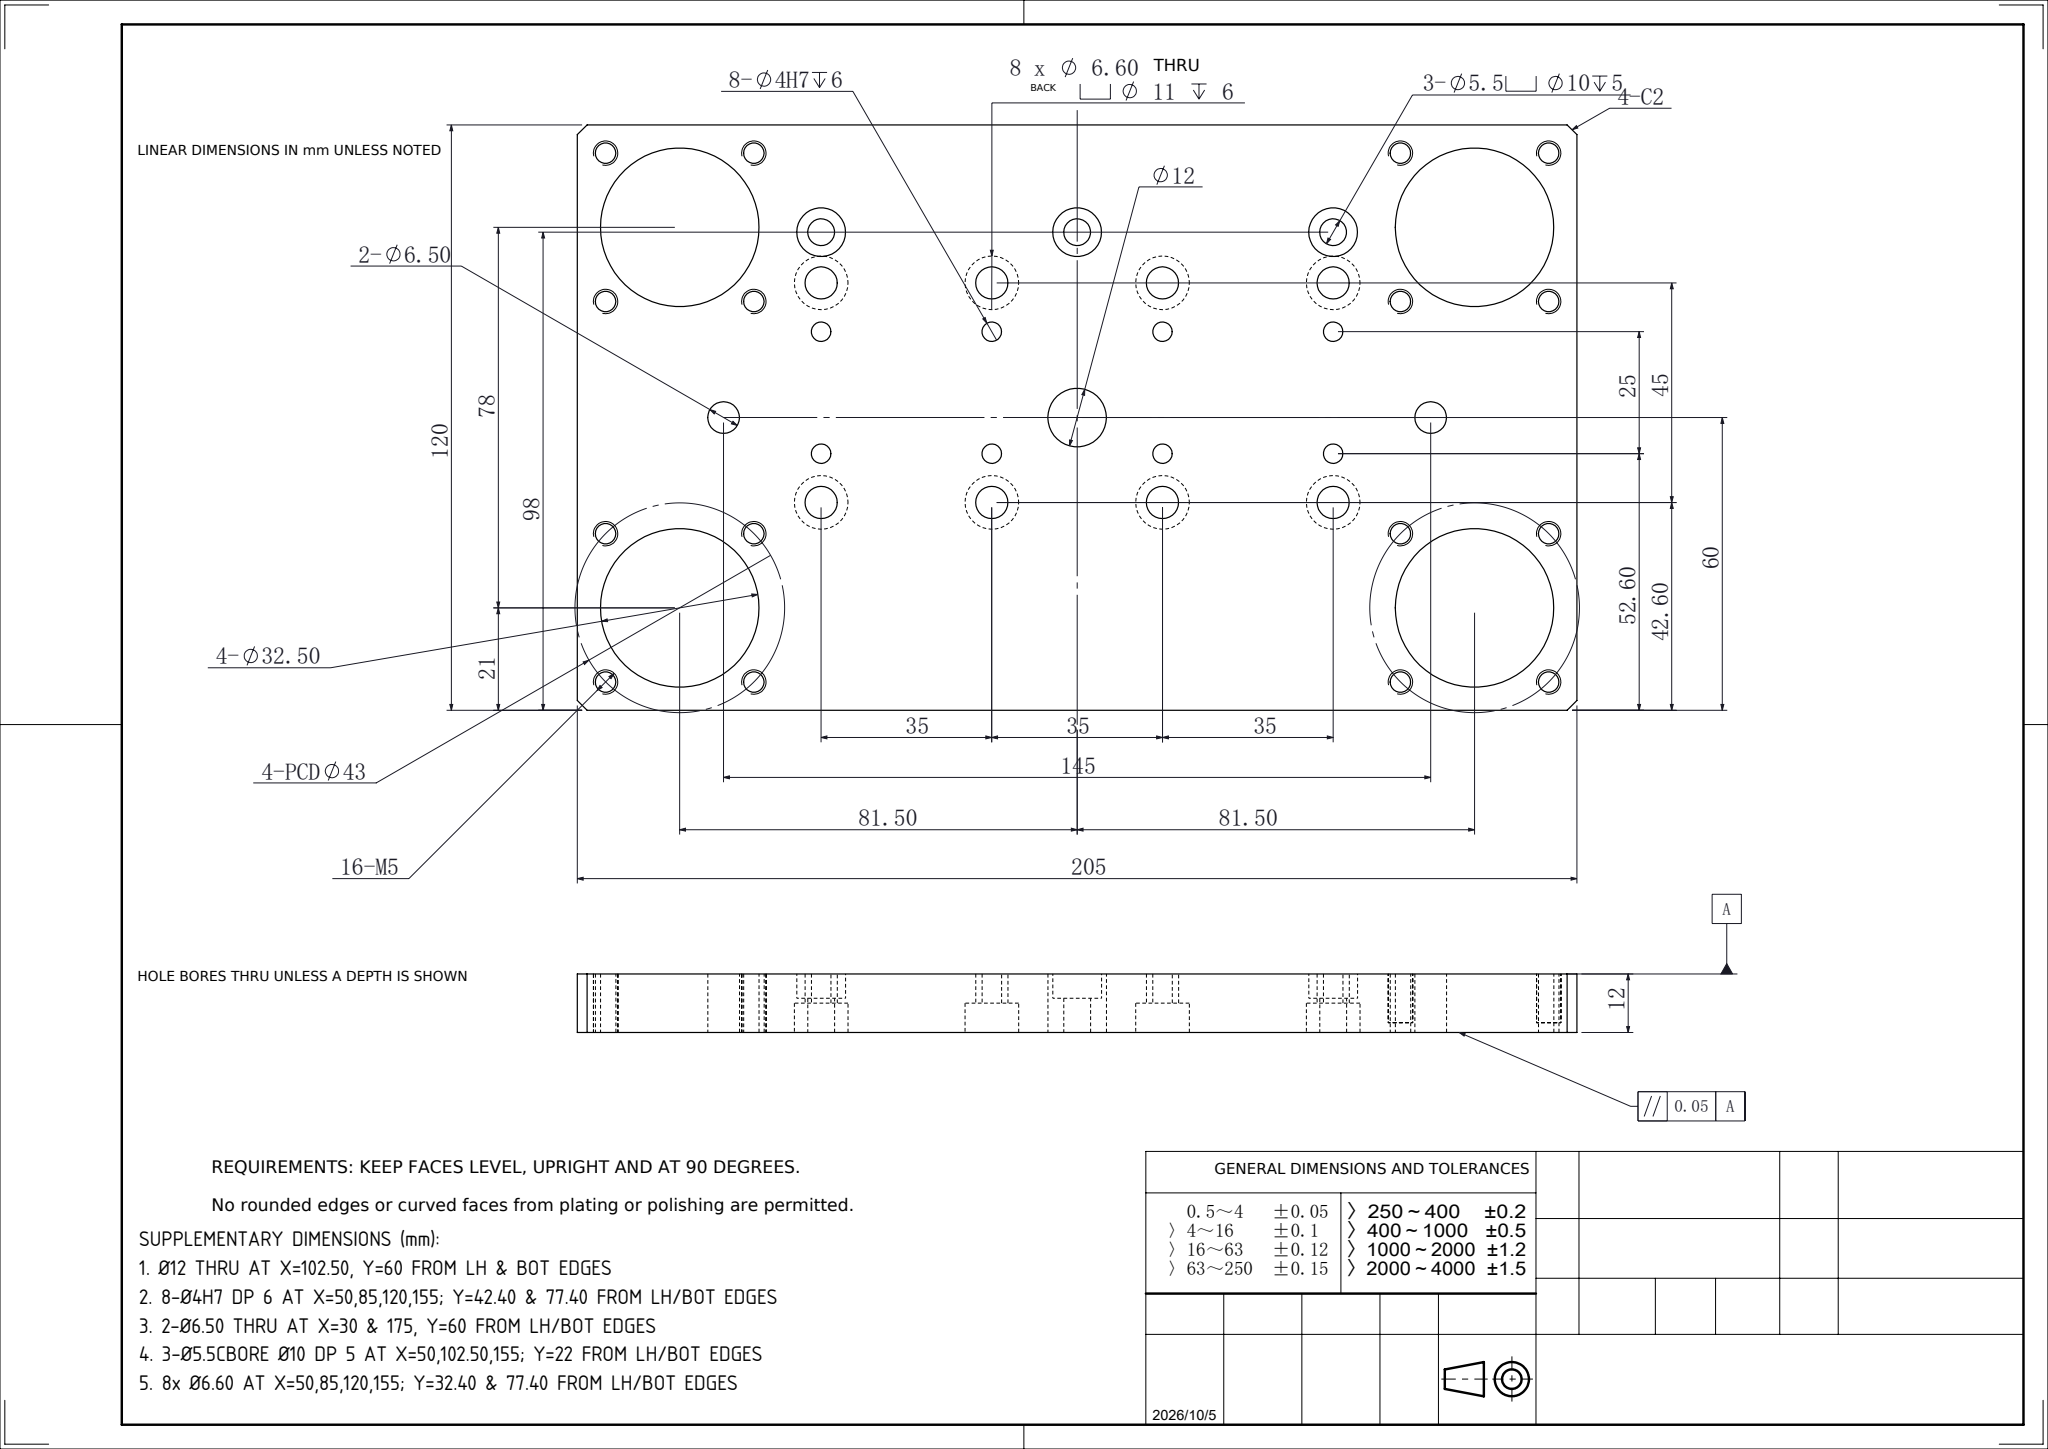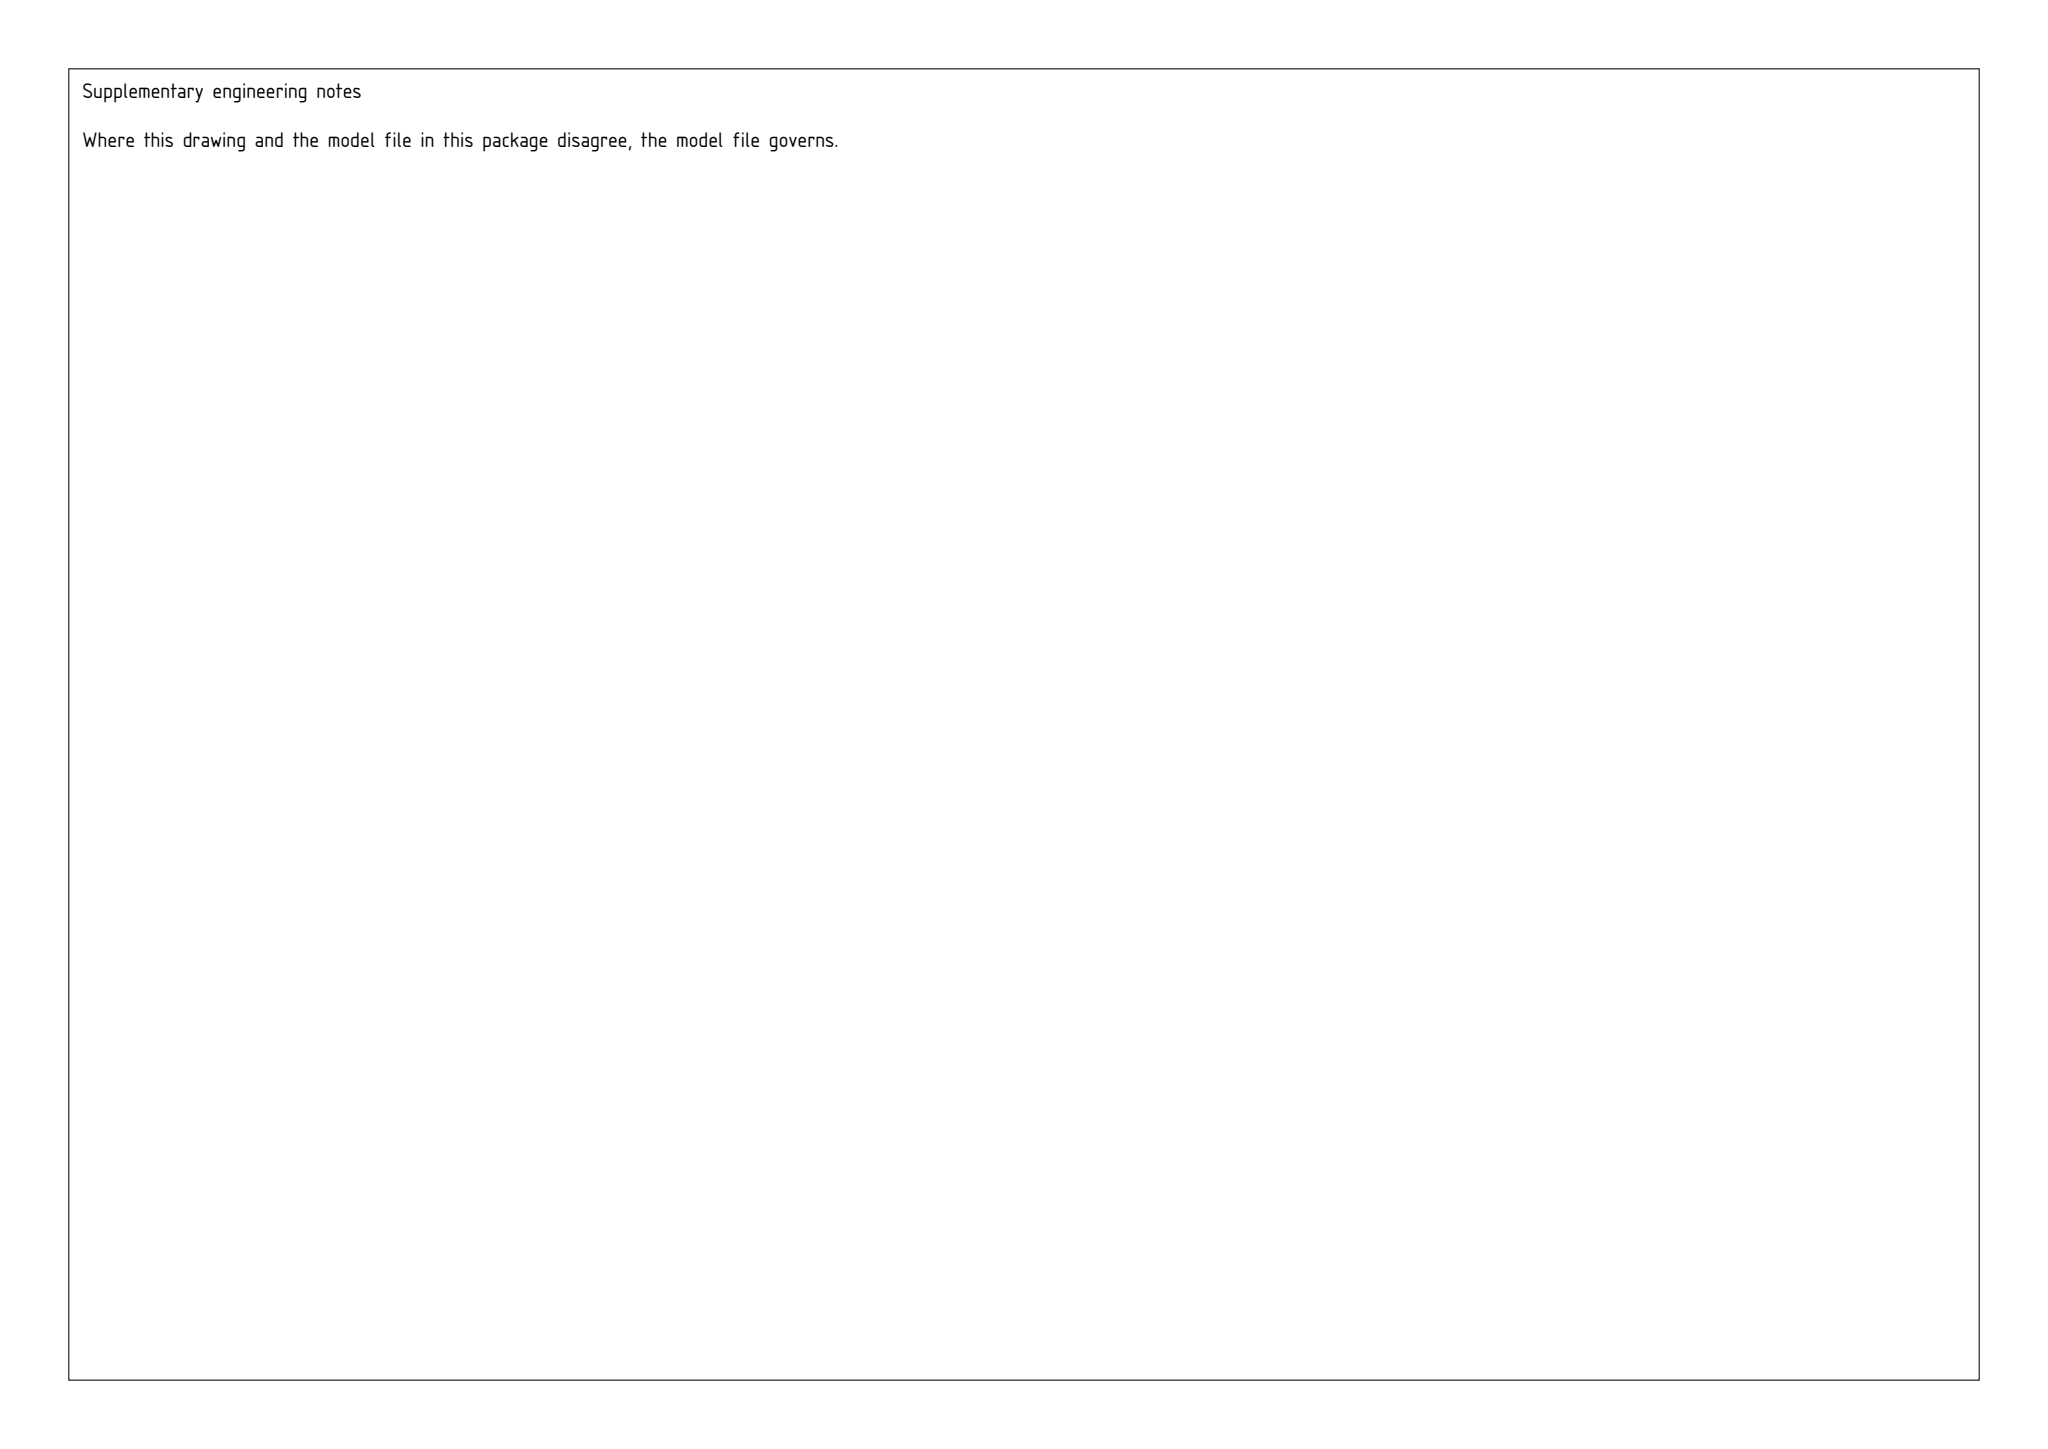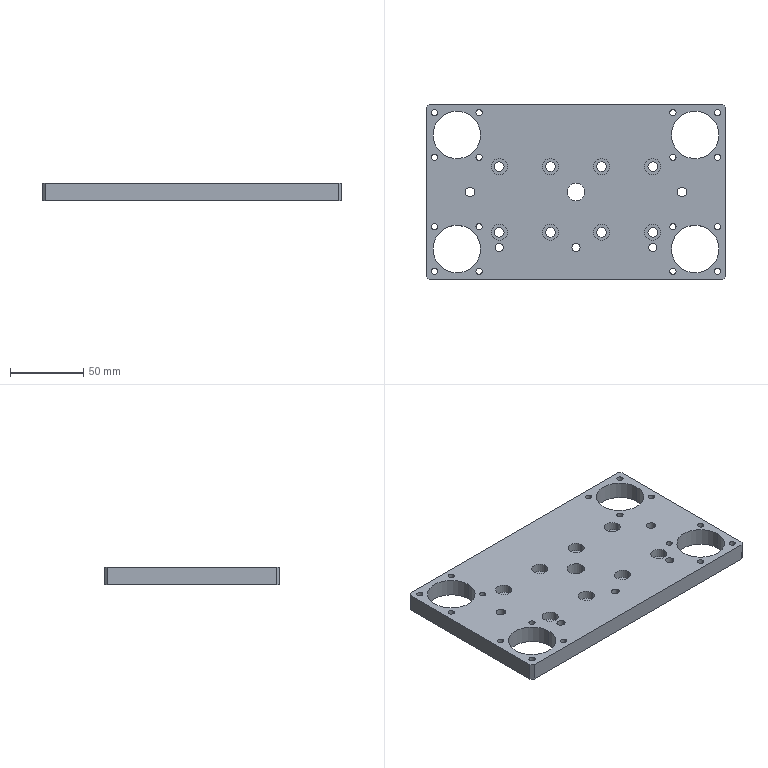Part | SolidWorks | mm | 1 solid | 135 faces | box 205 x 120 x 12 mm | volume 241987 mm3 | cylinder 106 | plane 29 | commonest cylinder face diameters 4.2 x32 4 x16 11 x16 6.6 x16 32.5 x8 10 x6 5.5 x6 6.5 x4
build123d program:
from build123d import *

# Parameters (mm, degrees)
SKETCH1_W                                       = 205
SKETCH1_H                                       = 120
BOSS_EXTRUDE1_DEPTH                             = 12
SKETCH8_R                                       = 16.25
CUT_EXTRUDE1_DEPTH                              = 159.273
M5_TAPPED_HOLE1_D                               = 4.2
CIRPATTERN1_COUNT                               = 4
CIRPATTERN2_COUNT                               = 4
SKETCH12_R                                      = 6
CUT_EXTRUDE2_DEPTH                              = 159.273
M6_HEX_SOCKET_HEAD_CAP_SCREW_CBORE2_D           = 6.6
M6_HEX_SOCKET_HEAD_CAP_SCREW_CBORE2_CBORE_D     = 11
M6_HEX_SOCKET_HEAD_CAP_SCREW_CBORE2_CBORE_DEPTH = 6
SKETCH14_R                                      = 2
CUT_EXTRUDE3_DEPTH                              = 6
CHAMFER1_SIZE                                   = 2
SKETCH20_R                                      = 3.25
CUT_EXTRUDE4_DEPTH                              = 159.273
M5_HEX_SOCKET_HEAD_CAP_SCREW_CBORE1_D           = 5.5
M5_HEX_SOCKET_HEAD_CAP_SCREW_CBORE1_CBORE_D     = 10
M5_HEX_SOCKET_HEAD_CAP_SCREW_CBORE1_CBORE_DEPTH = 5
LPATTERN1_COUNT                                 = 2
LPATTERN1_PITCH                                 = 78
LPATTERN1_COPY_1_D                              = 4.2
LPATTERN1_COPY_2_D                              = 4.2
LPATTERN1_COPY_3_D                              = 4.2


with BuildPart() as part:
    # Sketch1 → Boss-Extrude1 (new body)
    with BuildSketch(Plane.XY):
        with Locations((0, 60)):
            Rectangle(SKETCH1_W, SKETCH1_H)
    extrude(amount=BOSS_EXTRUDE1_DEPTH)

    # Sketch8 → Cut-Extrude1 (cut, through all)
    with BuildSketch(Plane(origin=(0, 0, 0), x_dir=(-1, 0, 0), z_dir=(0, 0, -1))):
        with Locations((-81.5, 99)):
            Circle(SKETCH8_R)
        with Locations((81.5, 99)):
            Circle(SKETCH8_R)
        with Locations((-81.5, 21)):
            Circle(SKETCH8_R)
        with Locations((81.5, 21)):
            Circle(SKETCH8_R)
    extrude(amount=-CUT_EXTRUDE1_DEPTH, mode=Mode.SUBTRACT)

    # M5 Tapped Hole1 (through all)
    with Locations(Plane(origin=(-96.703, 114.203, 0), x_dir=(-1, 0, 0), z_dir=(0, 0, -1))):
        with Locations((0, 0)):
            m5_tapped_hole1 = Hole(M5_TAPPED_HOLE1_D / 2)

    # Sketch11 → M5 Tapped Hole2 (revolve, cut)
    with BuildSketch(Plane(origin=(66.297, 114.203, 0), x_dir=(0, 1, 0), z_dir=(1, 0, 0))):
        Polygon((0, 0), (0, 17.262), (2.1, 16), (2.1, 0), align=None)
    m5_tapped_hole2 = revolve(axis=Axis((66.297, 114.203, -6.35), (0, 0, 1)), mode=Mode.SUBTRACT)

    # CirPattern1: M5 Tapped Hole1 ×4 about axis
    cirpattern1_axis = Axis((-81.5, 99, 0), (0, 0, 1))
    for i in range(1, CIRPATTERN1_COUNT):
        add(m5_tapped_hole1.rotate(cirpattern1_axis, i * 360 / CIRPATTERN1_COUNT), mode=Mode.SUBTRACT)

    # CirPattern2: M5 Tapped Hole2 ×4 about axis
    cirpattern2_axis = Axis((81.5, 99, 0), (0, 0, 1))
    for i in range(1, CIRPATTERN2_COUNT):
        add(m5_tapped_hole2.rotate(cirpattern2_axis, i * 360 / CIRPATTERN2_COUNT), mode=Mode.SUBTRACT)

    # Sketch12 → Cut-Extrude2 (cut, through all)
    with BuildSketch(Plane.XY.offset(12)):
        with Locations((0, 60)):
            Circle(SKETCH12_R)
    extrude(amount=-CUT_EXTRUDE2_DEPTH, mode=Mode.SUBTRACT)

    # M6 Hex Socket Head Cap Screw CBORE2 (through all)
    with Locations(Plane(origin=(-17.5, 77.4, 12), x_dir=(1, 0, 0), z_dir=(0, 0, 1))):
        with Locations((0, 0), (0, -45), (35, 0), (35, -45), (70, 0), (70, -45), (-35, 0), (-35, -45)):
            CounterBoreHole(M6_HEX_SOCKET_HEAD_CAP_SCREW_CBORE2_D / 2, M6_HEX_SOCKET_HEAD_CAP_SCREW_CBORE2_CBORE_D / 2, M6_HEX_SOCKET_HEAD_CAP_SCREW_CBORE2_CBORE_DEPTH)

    # Sketch14 → Cut-Extrude3 (cut)
    with BuildSketch(Plane.XY):
        with Locations((-17.5, 67.4)):
            Circle(SKETCH14_R)
        with Locations((-17.5, 42.4)):
            Circle(SKETCH14_R)
        with Locations((17.5, 67.4)):
            Circle(SKETCH14_R)
        with Locations((17.5, 42.4)):
            Circle(SKETCH14_R)
        with Locations((52.5, 67.4)):
            Circle(SKETCH14_R)
        with Locations((52.5, 42.4)):
            Circle(SKETCH14_R)
        with Locations((-52.5, 67.4)):
            Circle(SKETCH14_R)
        with Locations((-52.5, 42.4)):
            Circle(SKETCH14_R)
    extrude(amount=CUT_EXTRUDE3_DEPTH, mode=Mode.SUBTRACT)

    # Chamfer1
    chamfer1_edges = [part.edges().sort_by_distance(p)[0] for p in [
        (-102.5, 120, 6),
        (102.5, 120, 6),
        (102.5, 0, 6),
        (-102.5, 0, 6),
    ]]
    chamfer(chamfer1_edges, length=CHAMFER1_SIZE)

    # Sketch20 → Cut-Extrude4 (cut, through all)
    with BuildSketch(Plane(origin=(0, 0, 0), x_dir=(-1, 0, 0), z_dir=(0, 0, -1))):
        with Locations((72.5, 60)):
            Circle(SKETCH20_R)
        with Locations((-72.5, 60)):
            Circle(SKETCH20_R)
    extrude(amount=-CUT_EXTRUDE4_DEPTH, mode=Mode.SUBTRACT)

    # M5 Hex Socket Head Cap Screw CBORE1 (through all)
    with Locations(Plane(origin=(0, 0, 0), x_dir=(-1, 0, 0), z_dir=(0, 0, -1))):
        with Locations((52.5, 22), (0, 22), (-52.5, 22)):
            CounterBoreHole(M5_HEX_SOCKET_HEAD_CAP_SCREW_CBORE1_D / 2, M5_HEX_SOCKET_HEAD_CAP_SCREW_CBORE1_CBORE_D / 2, M5_HEX_SOCKET_HEAD_CAP_SCREW_CBORE1_CBORE_DEPTH)

    # LPattern1: M5 Tapped Hole1, M5 Tapped Hole2 ×2
    with Locations(*[(0, -i * LPATTERN1_PITCH, 0) for i in range(1, LPATTERN1_COUNT)]):
        add(m5_tapped_hole1, mode=Mode.SUBTRACT)
        add(m5_tapped_hole2, mode=Mode.SUBTRACT)

    # LPattern1 copy 1 (through all)
    with Locations(Plane(origin=(-96.703, 5.797, 0), x_dir=(0, -1, 0), z_dir=(0, 0, -1))):
        with Locations((0, 0)):
            Hole(LPATTERN1_COPY_1_D / 2)

    # LPattern1 copy 2 (through all)
    with Locations(Plane(origin=(-66.297, 5.797, 0), x_dir=(1, 0, 0), z_dir=(0, 0, -1))):
        with Locations((0, 0)):
            Hole(LPATTERN1_COPY_2_D / 2)

    # LPattern1 copy 3 (through all)
    with Locations(Plane(origin=(-66.297, 36.203, 0), x_dir=(0, 1, 0), z_dir=(0, 0, -1))):
        with Locations((0, 0)):
            Hole(LPATTERN1_COPY_3_D / 2)

    # LPattern1 copy 4 sketch → LPattern1 copy 4 (revolve, cut)
    with BuildSketch(Plane(origin=(66.297, 5.797, 0), x_dir=(-1, 0, 0), z_dir=(0, 1, 0))):
        Polygon((0, 0), (0, 17.262), (2.1, 16), (2.1, 0), align=None)
    revolve(axis=Axis((66.297, 5.797, -6.35), (0, 0, 1)), mode=Mode.SUBTRACT)

    # LPattern1 copy 5 sketch → LPattern1 copy 5 (revolve, cut)
    with BuildSketch(Plane(origin=(96.703, 5.797, 0), x_dir=(0, -1, 0), z_dir=(-1, 0, 0))):
        Polygon((0, 0), (0, 17.262), (2.1, 16), (2.1, 0), align=None)
    revolve(axis=Axis((96.703, 5.797, -6.35), (0, 0, 1)), mode=Mode.SUBTRACT)

    # LPattern1 copy 6 sketch → LPattern1 copy 6 (revolve, cut)
    with BuildSketch(Plane(origin=(96.703, 36.203, 0), x_dir=(1, 0, 0), z_dir=(0, -1, 0))):
        Polygon((0, 0), (0, 17.262), (2.1, 16), (2.1, 0), align=None)
    revolve(axis=Axis((96.703, 36.203, -6.35), (0, 0, 1)), mode=Mode.SUBTRACT)


solid = part.part